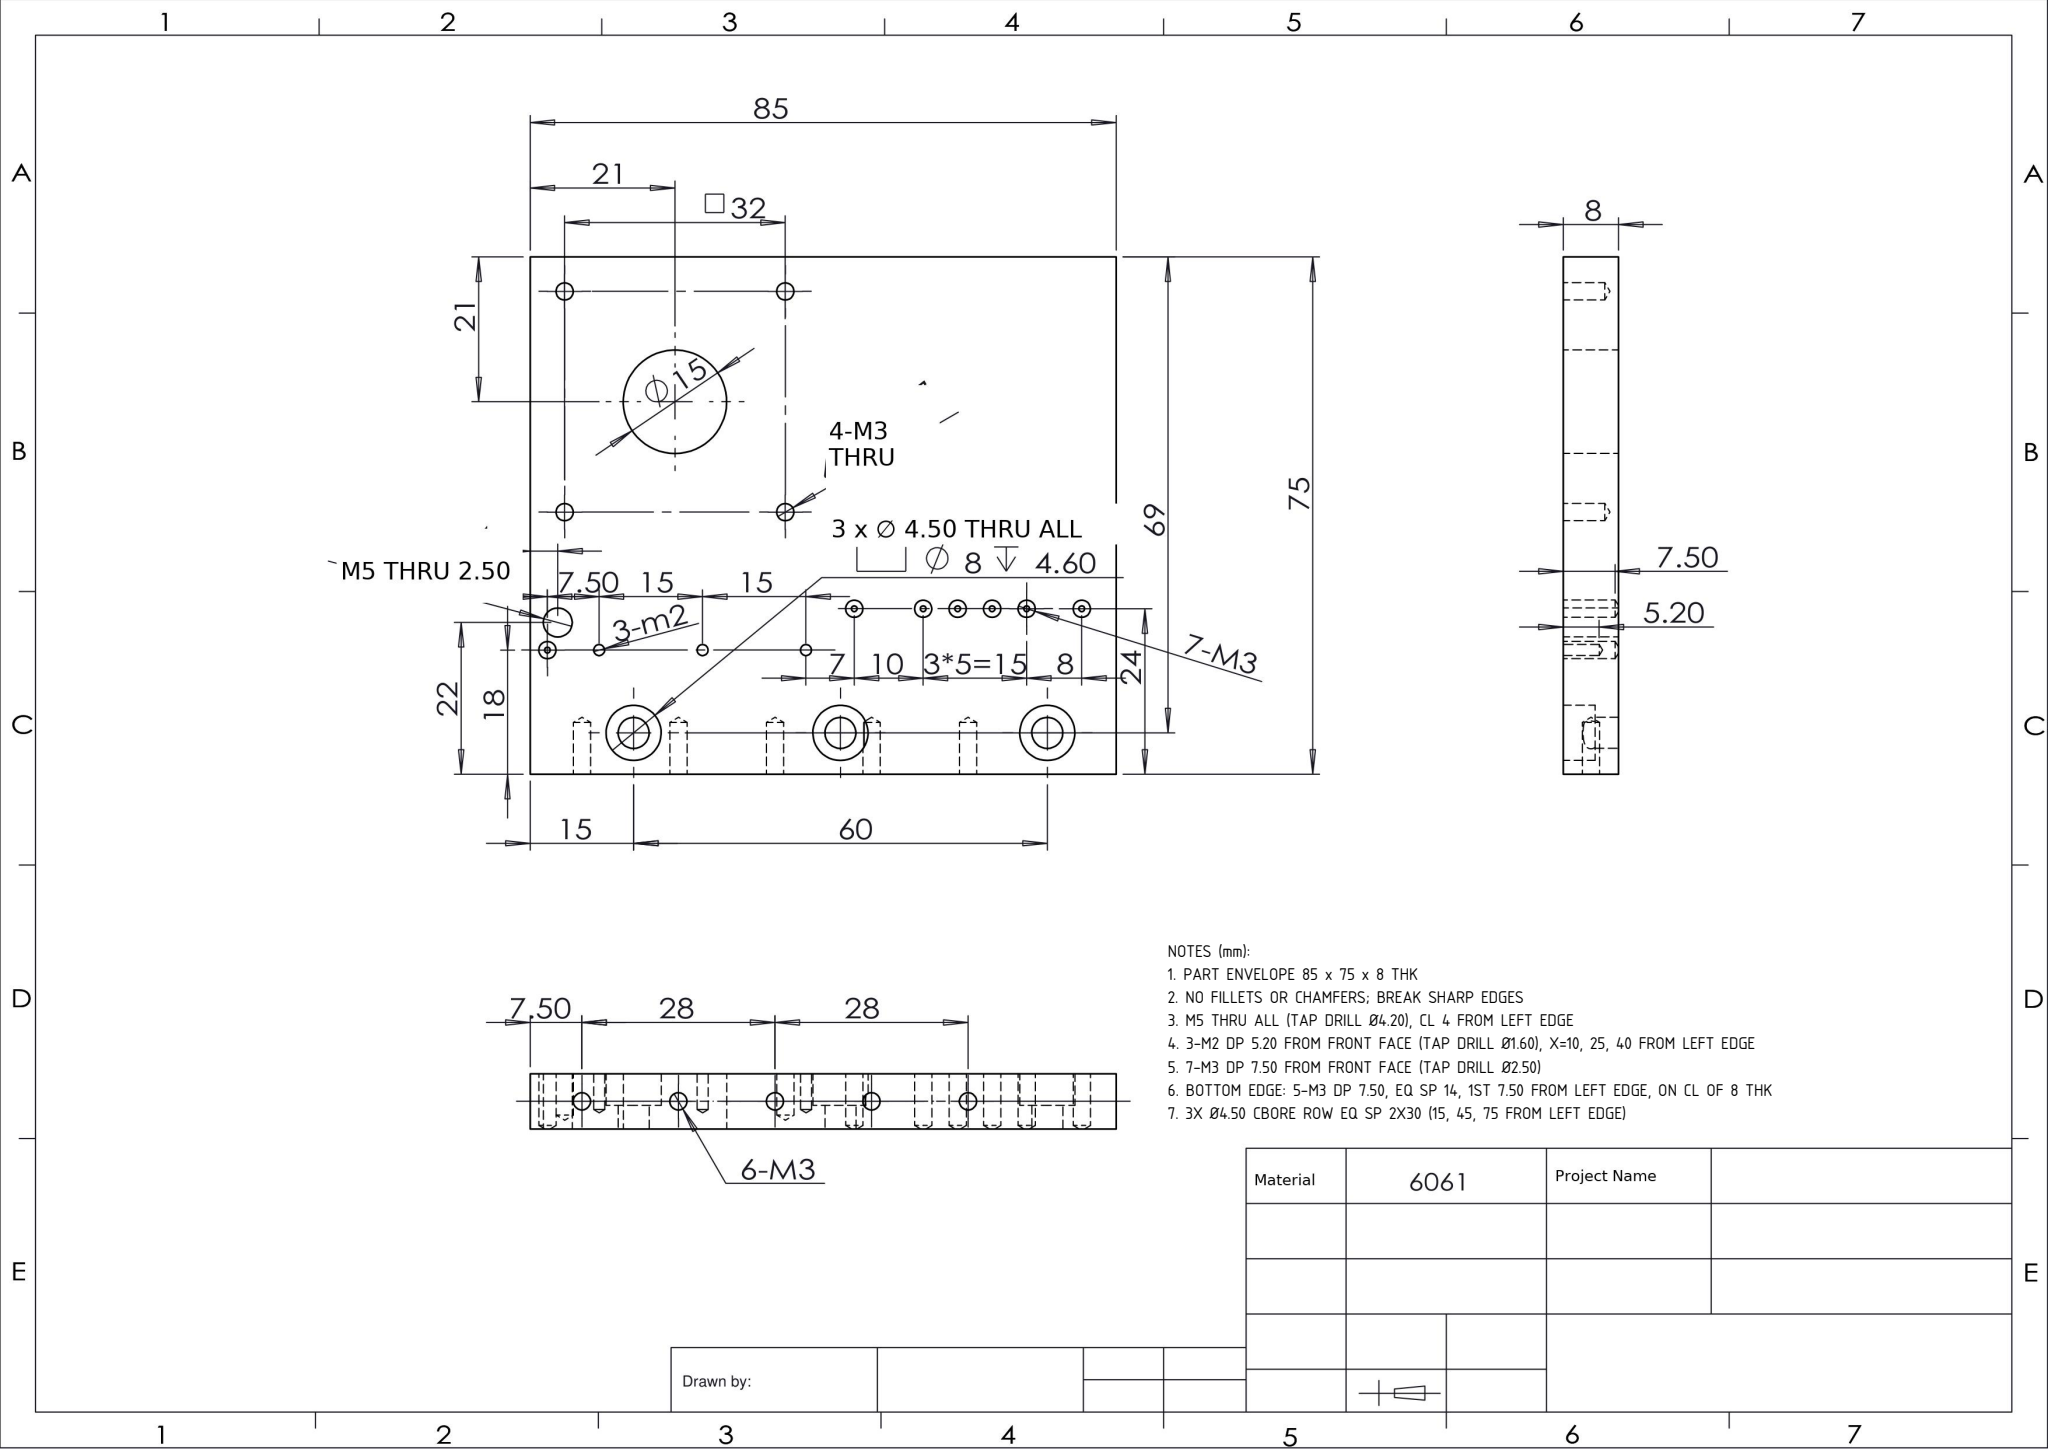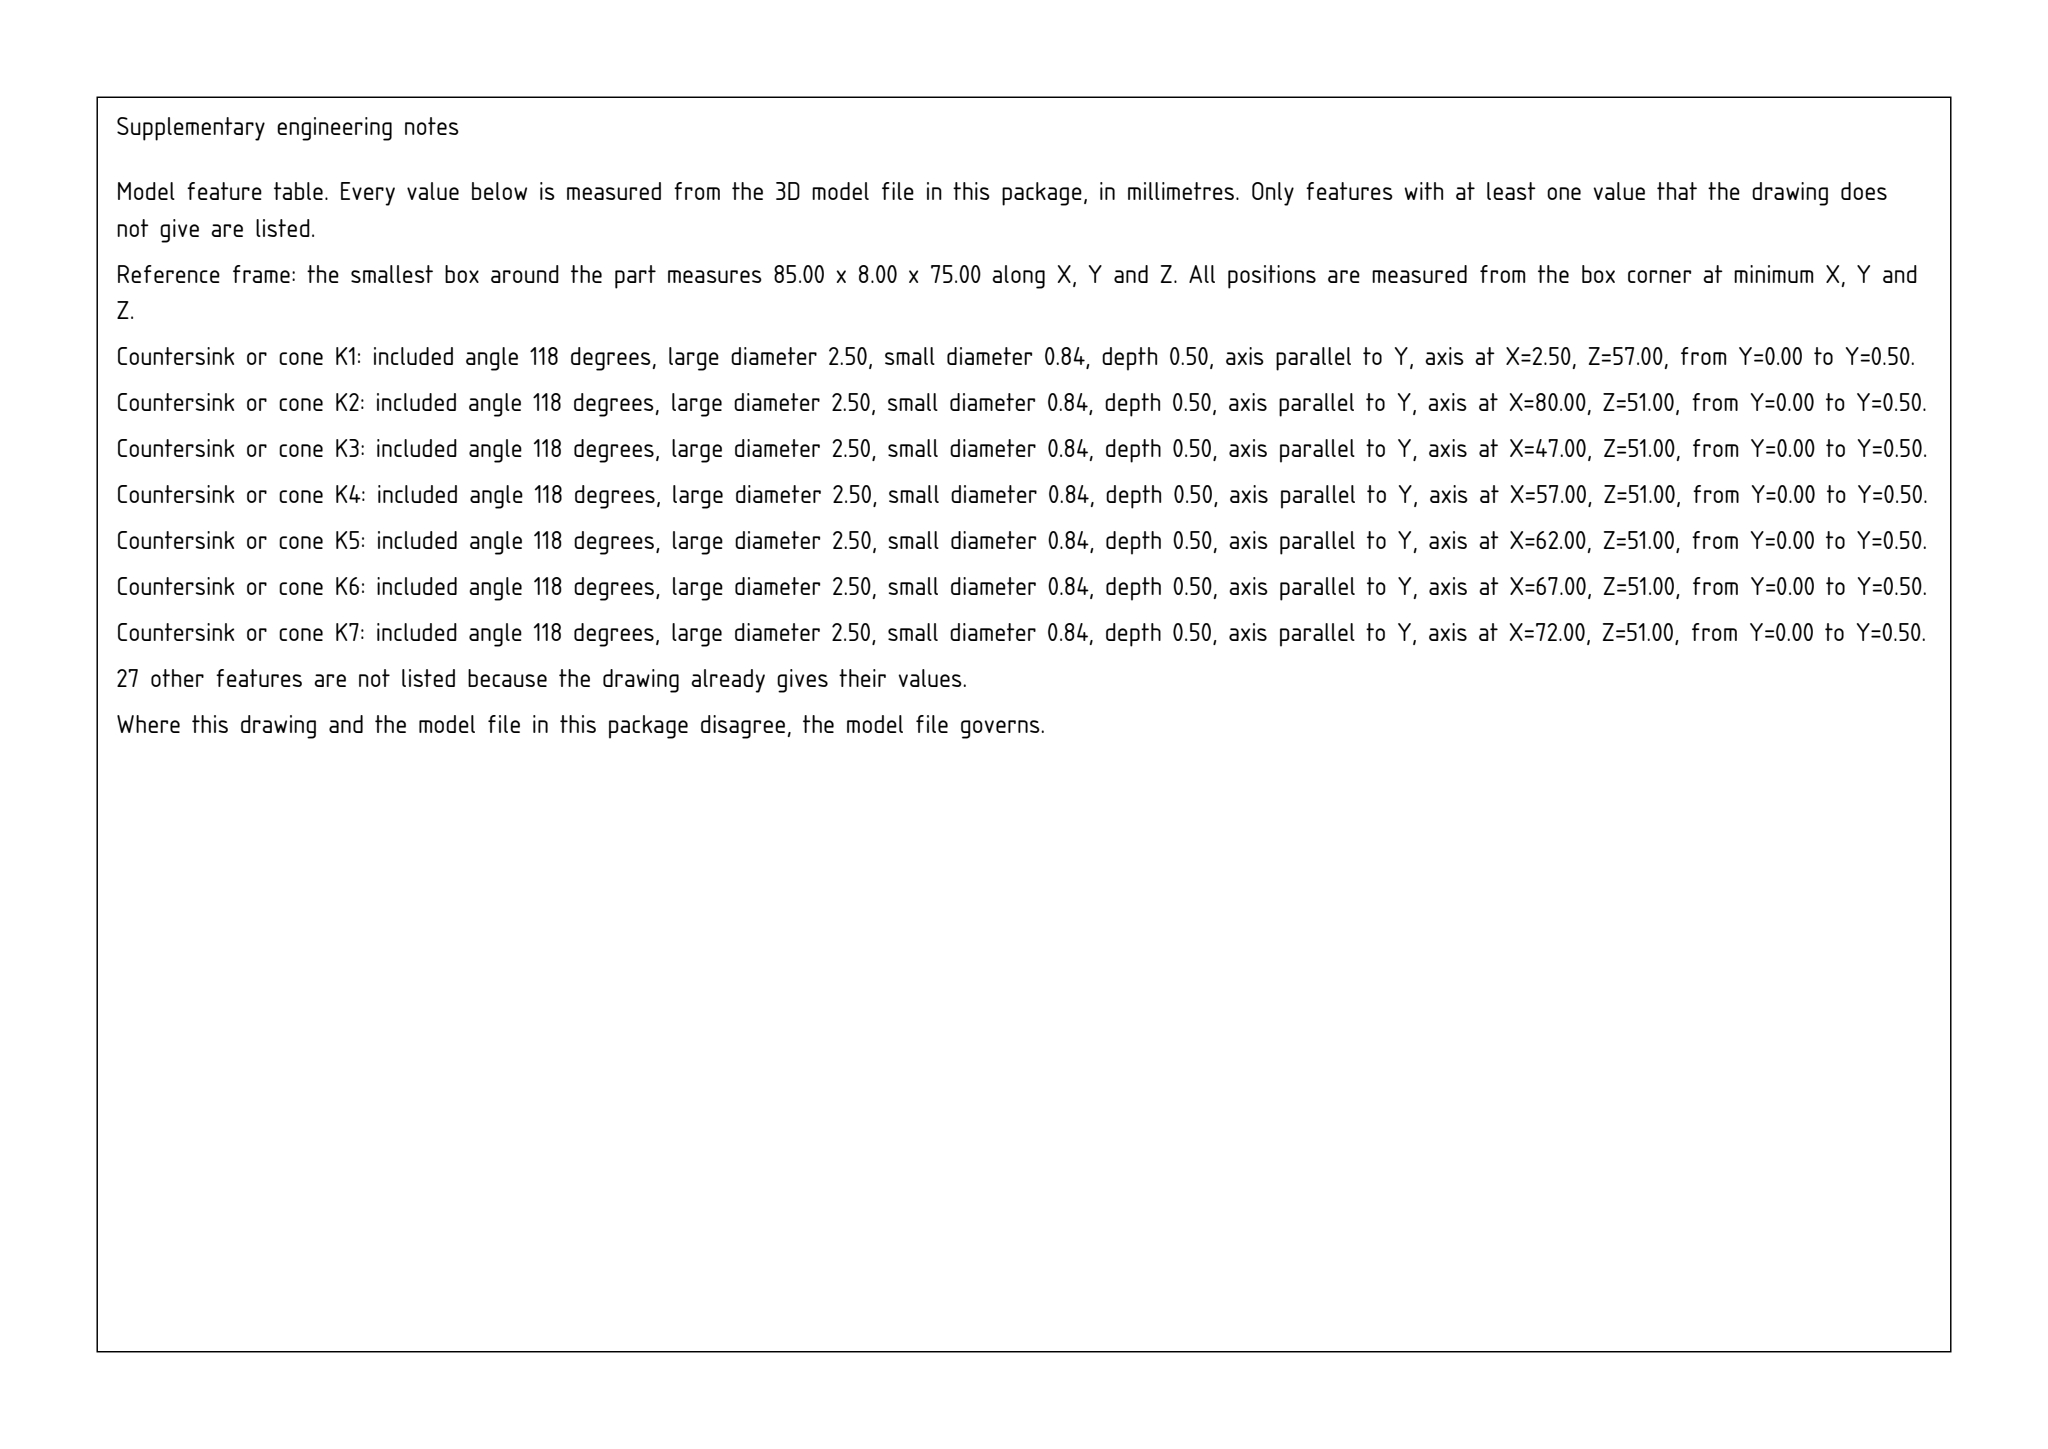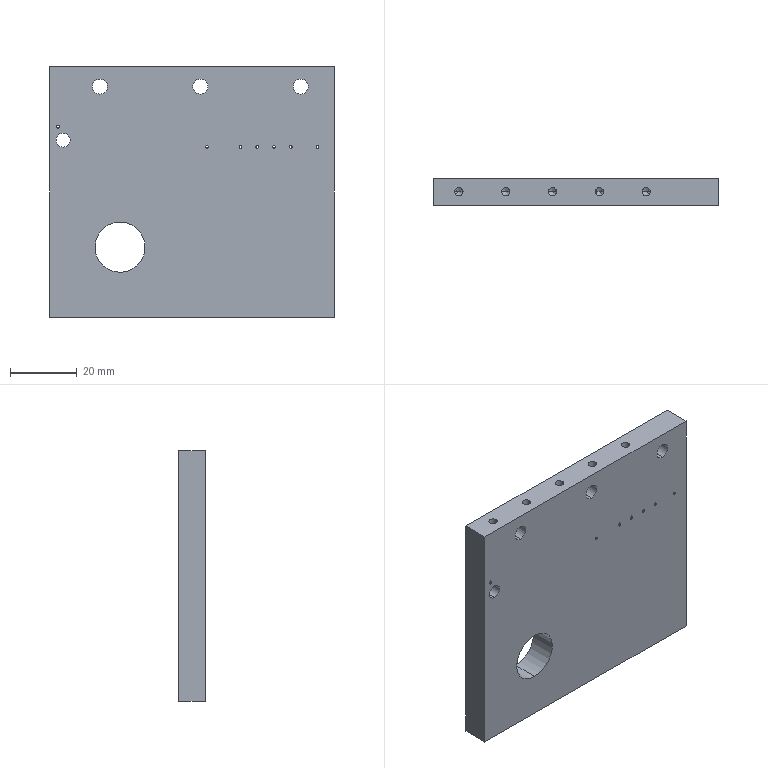Part | SolidWorks | mm | 1 solid | 101 faces | box 85 x 8 x 75 mm | volume 48011 mm3 | cylinder 54 | cone 38 | plane 9 | commonest cylinder face diameters 2.5 x32 1.6 x6 8 x6 4.5 x6 4.2 x2 15 x2
Drawing notes:
PART ENVELOPE 85 x 75 x 8 THK | from the solid: bbox_xyz [85.0, 8.0, 75.0]
NO FILLETS OR CHAMFERS; BREAK SHARP EDGES | from the solid: fillet_radii empty; only 118° drill point cones present
M5 THRU ALL (TAP DRILL Ø4.20), CL 4 FROM LEFT EDGE | from the solid: Ø4.2 y-axis cyl, L=8.0 (full thk), x=4.0, z=53 (75-53=22)
3-M2 DP 5.20 FROM FRONT FACE (TAP DRILL Ø1.60), X=10, 25, 40 FROM LEFT EDGE | from the solid: Ø1.6 y-axis cyls L=5.2 at (10,57),(25,57),(40,57); 118° points ref Ø1.6; 75-57=18
7-M3 DP 7.50 FROM FRONT FACE (TAP DRILL Ø2.50) | from the solid: Ø2.5 y-axis cyls L=7.5 at (2.5,57) and (47/57/62/67/72/80, 51) = 7 PL
BOTTOM EDGE: 5-M3 DP 7.50, EQ SP 14, 1ST 7.50 FROM LEFT EDGE, ON CL OF 8 THK | from the solid: Ø2.5 z-axis cyls L=7.5, y=4.0, x=7.5/21.5/35.5/49.5/63.5
3X Ø4.50 CBORE ROW EQ SP 2X30 (15, 45, 75 FROM LEFT EDGE) | from the solid: Ø4.5/Ø8 cbore cylinders at x=15, 45, 75, z=69 — equal 30 spacing
build123d program:
from build123d import *

# Parameters (mm, degrees)
SKETCH1_W                                            = 85
SKETCH1_H                                            = 8
BOSS_EXTRUDE1_DEPTH                                  = 37.5
HOLE_SIZE_ACCORDING_TO_THE_TYPE_OF_HEXAG_D           = 4.5
HOLE_SIZE_ACCORDING_TO_THE_TYPE_OF_HEXAG_CBORE_D     = 8
HOLE_SIZE_ACCORDING_TO_THE_TYPE_OF_HEXAG_CBORE_DEPTH = 4.6
M3_TAPPED_HOLE1_D                                    = 2.5
M3_TAPPED_HOLE1_DEPTH                                = 6
M3_TAPPED_HOLE1_TIP                                  = 0.7511
SKETCH12_R                                           = 7.5
CUT_EXTRUDE1_DEPTH                                   = 58.241
LPATTERN1_COUNT                                      = 5
LPATTERN1_PITCH                                      = 14
M5_TAPPED_HOLE1_D                                    = 4.2
M5_TAPPED_HOLE1_DEPTH                                = 12.4
M5_TAPPED_HOLE1_TIP                                  = 1.262
M2_TAPPED_HOLE1_D                                    = 1.6
M2_TAPPED_HOLE1_DEPTH                                = 5.2
M2_TAPPED_HOLE1_TIP                                  = 0.4807
M3_TAPPED_HOLE3_D                                    = 2.5
M3_TAPPED_HOLE3_DEPTH                                = 7.5
M3_TAPPED_HOLE3_TIP                                  = 0.7511


with BuildPart() as part:
    # Sketch1 → Boss-Extrude1 (new, symmetric)
    with BuildSketch(Plane.XY):
        Rectangle(SKETCH1_W, SKETCH1_H)
    extrude(amount=BOSS_EXTRUDE1_DEPTH, both=True)

    # Hole Size according to the type of hexag (through all)
    with Locations(Plane(origin=(10.996, 4, 49.69), x_dir=(1, 0, 0), z_dir=(0, 1, 0))):
        with Locations((-38.496, 18.19), (-8.496, 18.19), (21.504, 18.19)):
            CounterBoreHole(HOLE_SIZE_ACCORDING_TO_THE_TYPE_OF_HEXAG_D / 2, HOLE_SIZE_ACCORDING_TO_THE_TYPE_OF_HEXAG_CBORE_D / 2, HOLE_SIZE_ACCORDING_TO_THE_TYPE_OF_HEXAG_CBORE_DEPTH)

    # M3 Tapped Hole1
    with Locations(Plane(origin=(-24.419, 4, -48.501), x_dir=(1, 0, 0), z_dir=(0, 1, 0))):
        with Locations((-13.081, -48.001), (18.919, -16.001), (-13.081, -16.001), (18.919, -48.001)):
            Hole(M3_TAPPED_HOLE1_D / 2, depth=M3_TAPPED_HOLE1_DEPTH)
            with Locations((0, 0, -(M3_TAPPED_HOLE1_DEPTH + M3_TAPPED_HOLE1_TIP / 2))):  # 118° drill point
                Cone(0, M3_TAPPED_HOLE1_D / 2, M3_TAPPED_HOLE1_TIP, mode=Mode.SUBTRACT)

    # Sketch12 → Cut-Extrude1 (cut, through all)
    with BuildSketch(Plane(origin=(0, 4, 0), x_dir=(1, 0, 0), z_dir=(0, 1, 0))):
        with Locations(Location((-21.5, 16.5, 0), (0, 0, 270))):
            Circle(SKETCH12_R)
    extrude(amount=-CUT_EXTRUDE1_DEPTH, mode=Mode.SUBTRACT)

    # Sketch13 → M3 Tapped Hole2 (revolve, cut)
    with BuildSketch(Plane(origin=(-35, 0, 37.5), x_dir=(0, -1, 0), z_dir=(1, 0, 0))):
        Polygon((0, 0), (0, 8.251), (1.25, 7.5), (1.25, 0), align=None)
    m3_tapped_hole2 = revolve(axis=Axis((-35, 0, 43.85), (0, 0, -1)), mode=Mode.SUBTRACT)

    # LPattern1: M3 Tapped Hole2 ×5
    with Locations(*[(i * LPATTERN1_PITCH, 0, 0) for i in range(1, LPATTERN1_COUNT)]):
        add(m3_tapped_hole2, mode=Mode.SUBTRACT)

    # M5 Tapped Hole1
    with Locations(Plane(origin=(0, 4, 0), x_dir=(1, 0, 0), z_dir=(0, 1, 0))):
        with Locations((-38.5, -15.5)):
            Hole(M5_TAPPED_HOLE1_D / 2, depth=M5_TAPPED_HOLE1_DEPTH)
            with Locations((0, 0, -(M5_TAPPED_HOLE1_DEPTH + M5_TAPPED_HOLE1_TIP / 2))):  # 118° drill point
                Cone(0, M5_TAPPED_HOLE1_D / 2, M5_TAPPED_HOLE1_TIP, mode=Mode.SUBTRACT)

    # M2 Tapped Hole1
    with Locations(Plane(origin=(0, 4, 0), x_dir=(1, 0, 0), z_dir=(0, 1, 0))):
        with Locations((-32.5, -19.5), (-17.5, -19.5), (-2.5, -19.5)):
            Hole(M2_TAPPED_HOLE1_D / 2, depth=M2_TAPPED_HOLE1_DEPTH)
            with Locations((0, 0, -(M2_TAPPED_HOLE1_DEPTH + M2_TAPPED_HOLE1_TIP / 2))):  # 118° drill point
                Cone(0, M2_TAPPED_HOLE1_D / 2, M2_TAPPED_HOLE1_TIP, mode=Mode.SUBTRACT)

    # M3 Tapped Hole3
    with Locations(Plane(origin=(0, 4, 0), x_dir=(1, 0, 0), z_dir=(0, 1, 0))):
        with Locations((4.5, -13.5), (-40, -19.5), (14.5, -13.5), (19.5, -13.5), (24.5, -13.5), (29.5, -13.5), (37.5, -13.5)):
            Hole(M3_TAPPED_HOLE3_D / 2, depth=M3_TAPPED_HOLE3_DEPTH)
            with Locations((0, 0, -(M3_TAPPED_HOLE3_DEPTH + M3_TAPPED_HOLE3_TIP / 2))):  # 118° drill point
                Cone(0, M3_TAPPED_HOLE3_D / 2, M3_TAPPED_HOLE3_TIP, mode=Mode.SUBTRACT)


solid = part.part